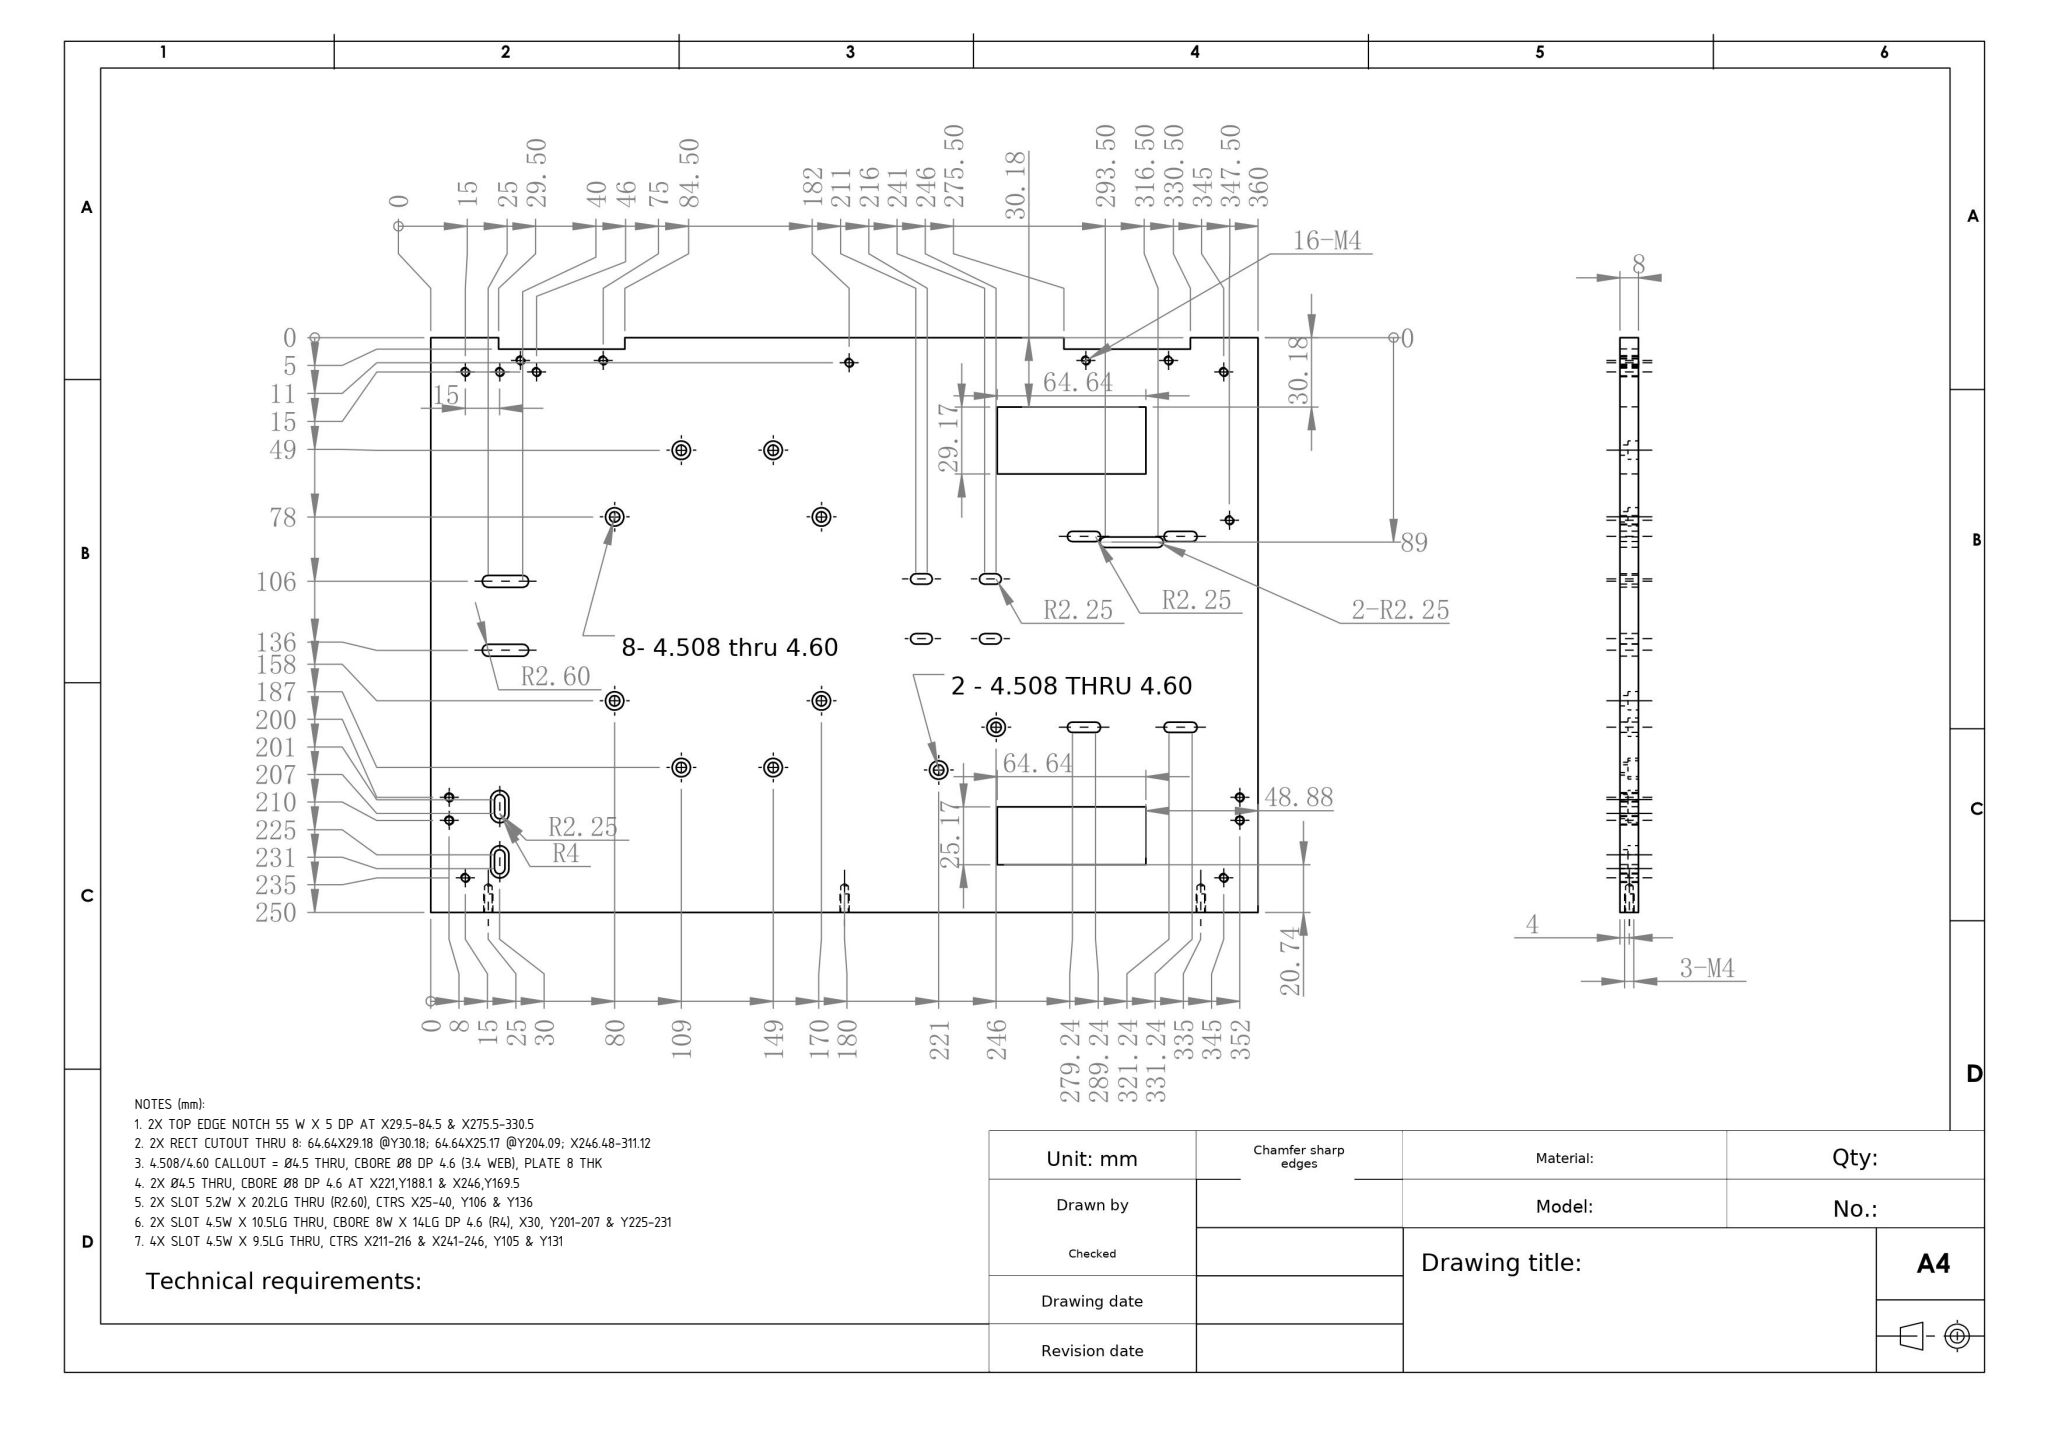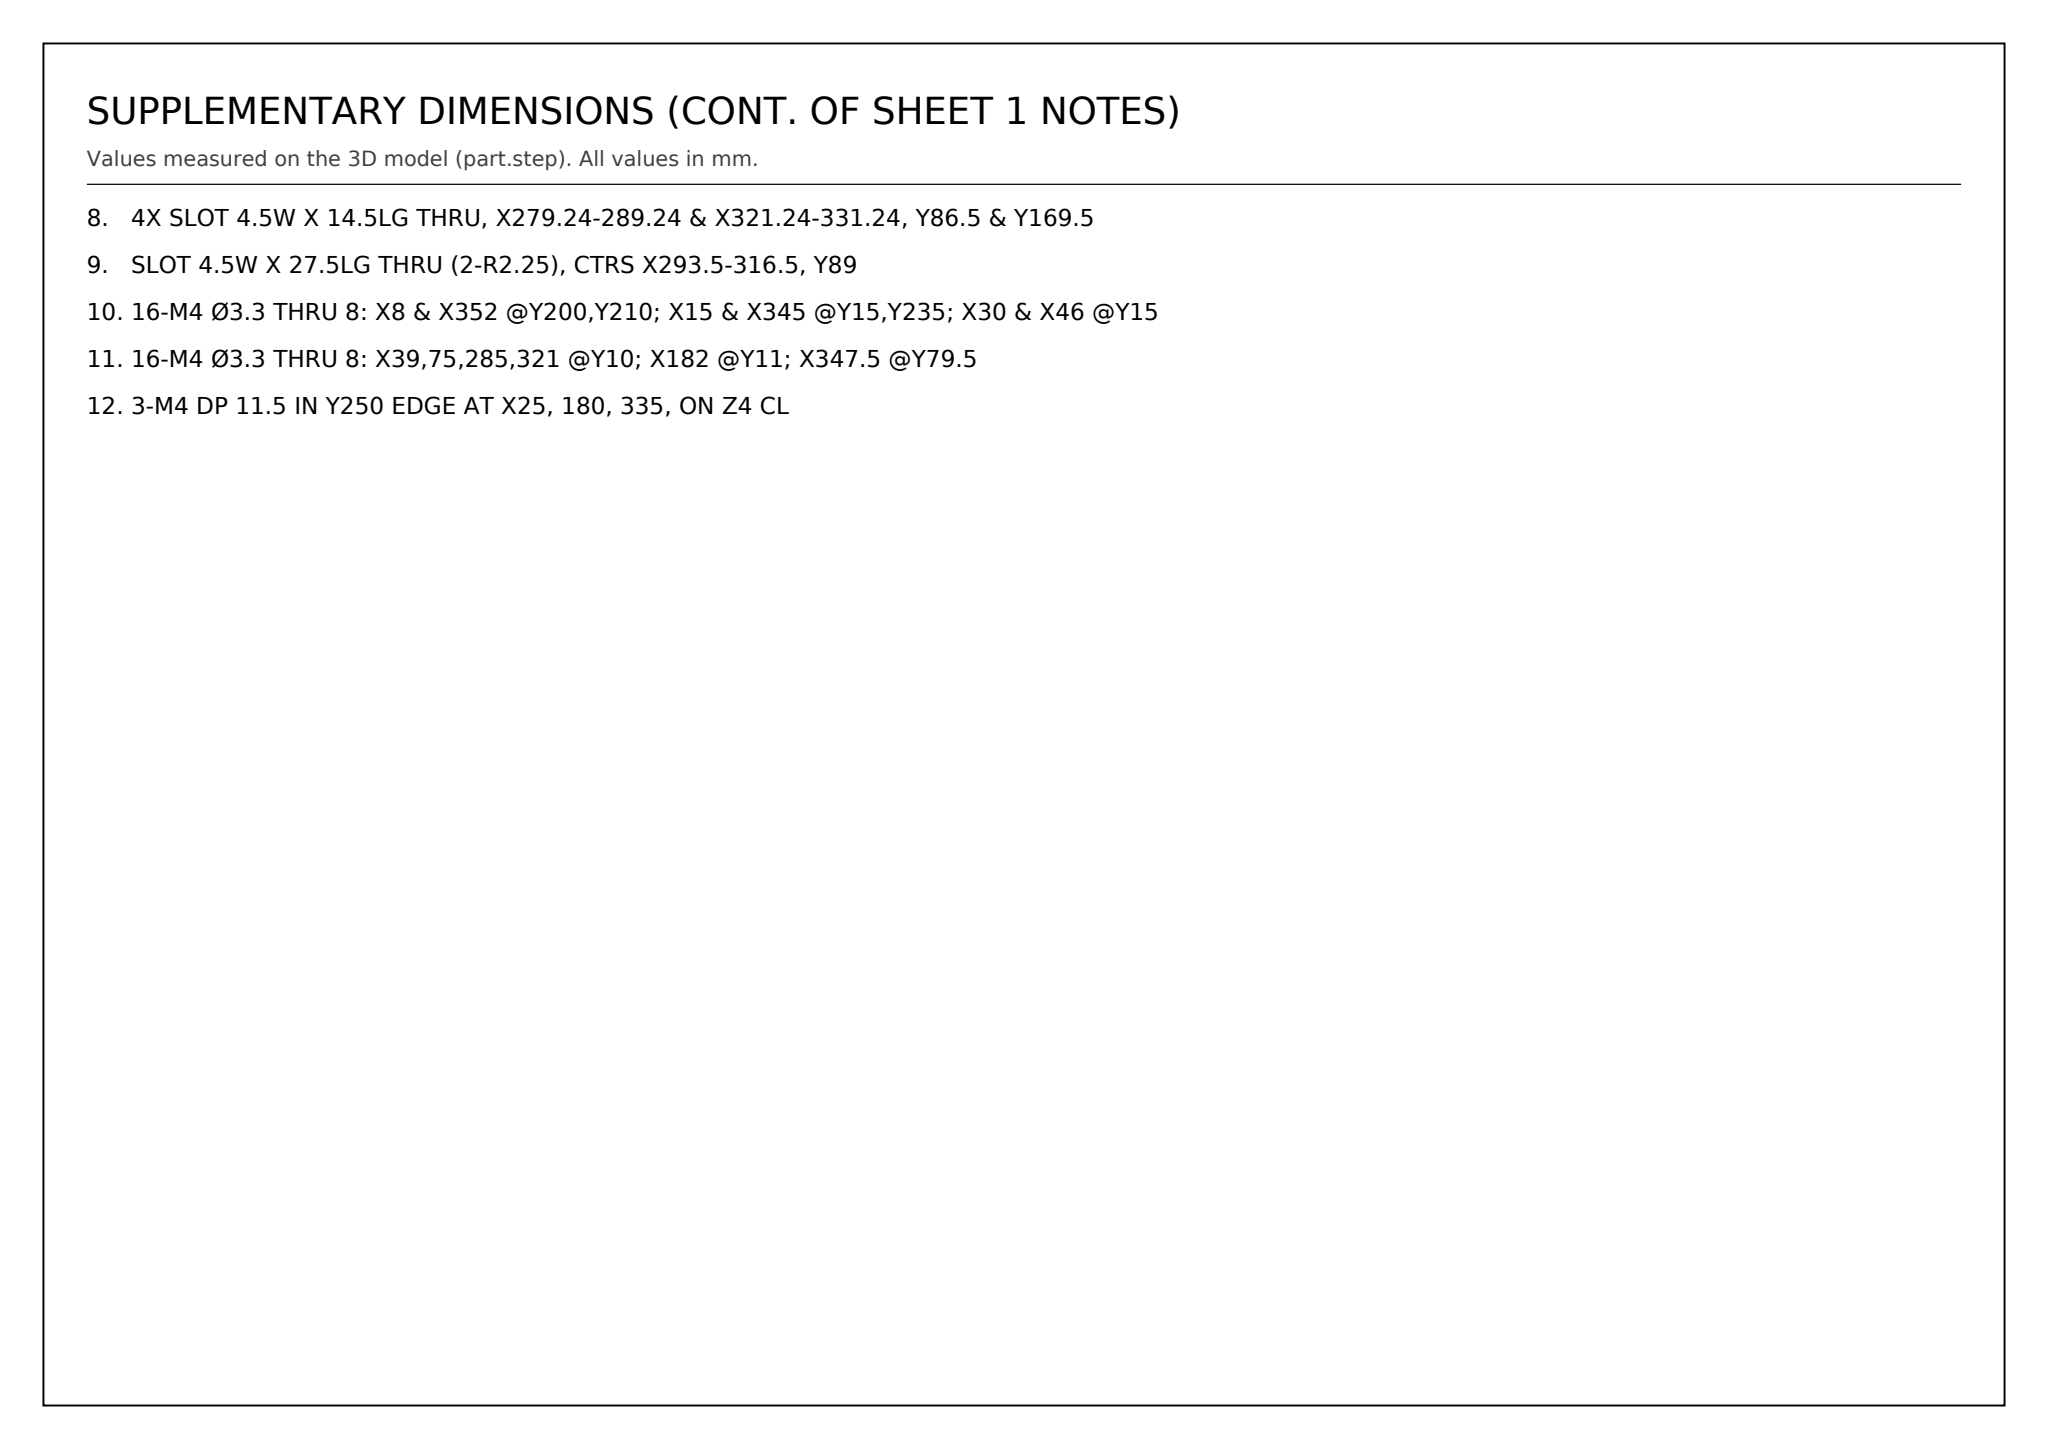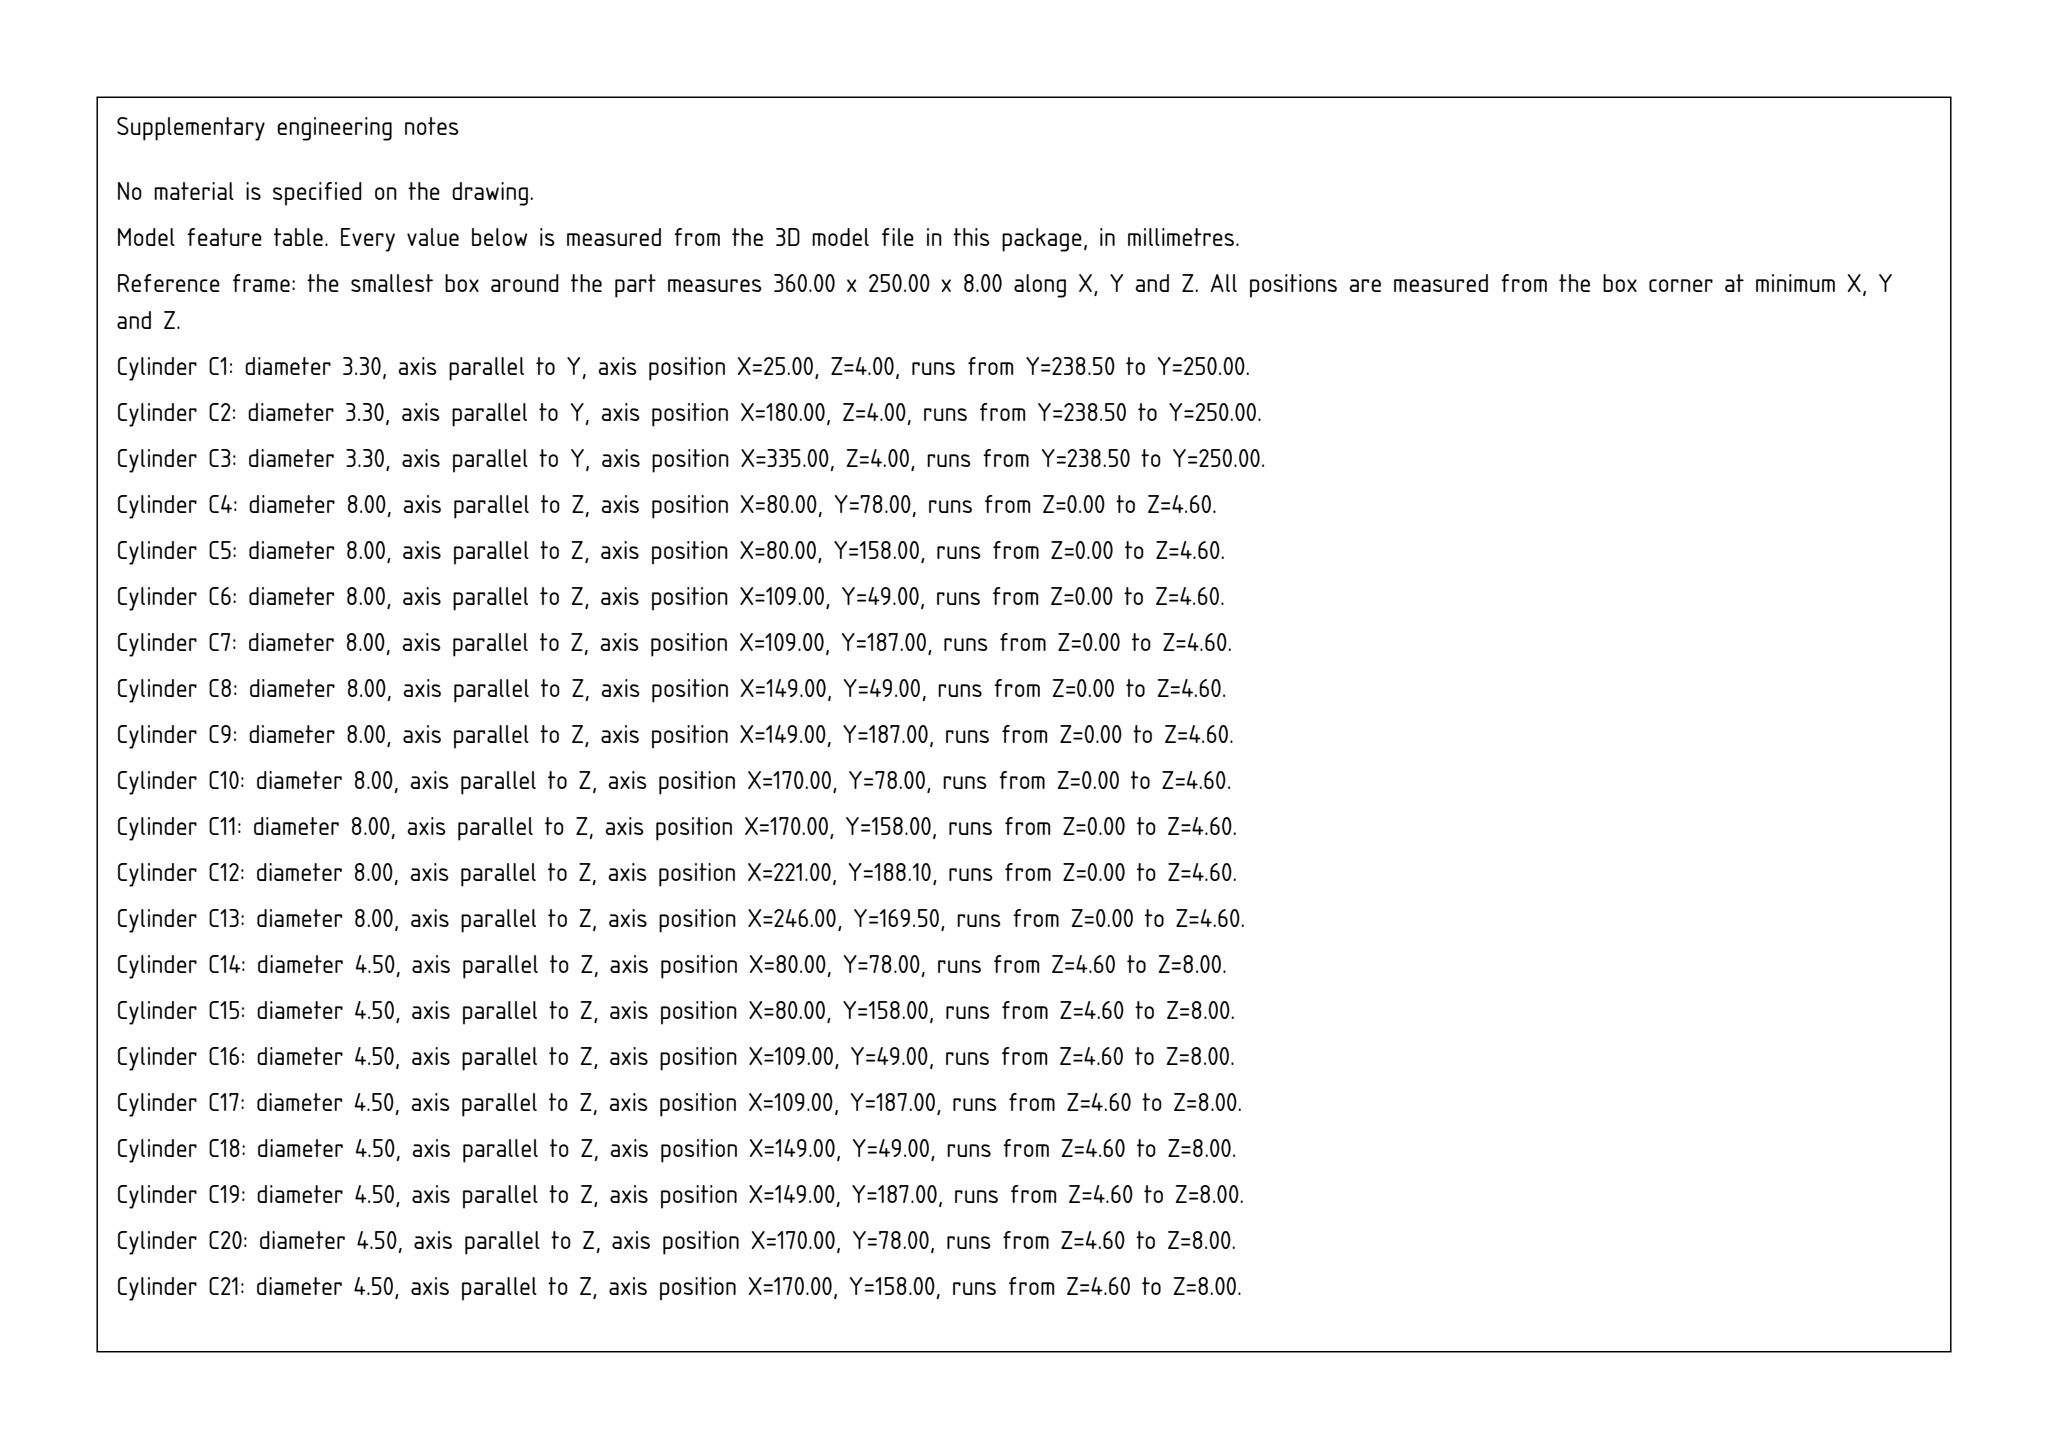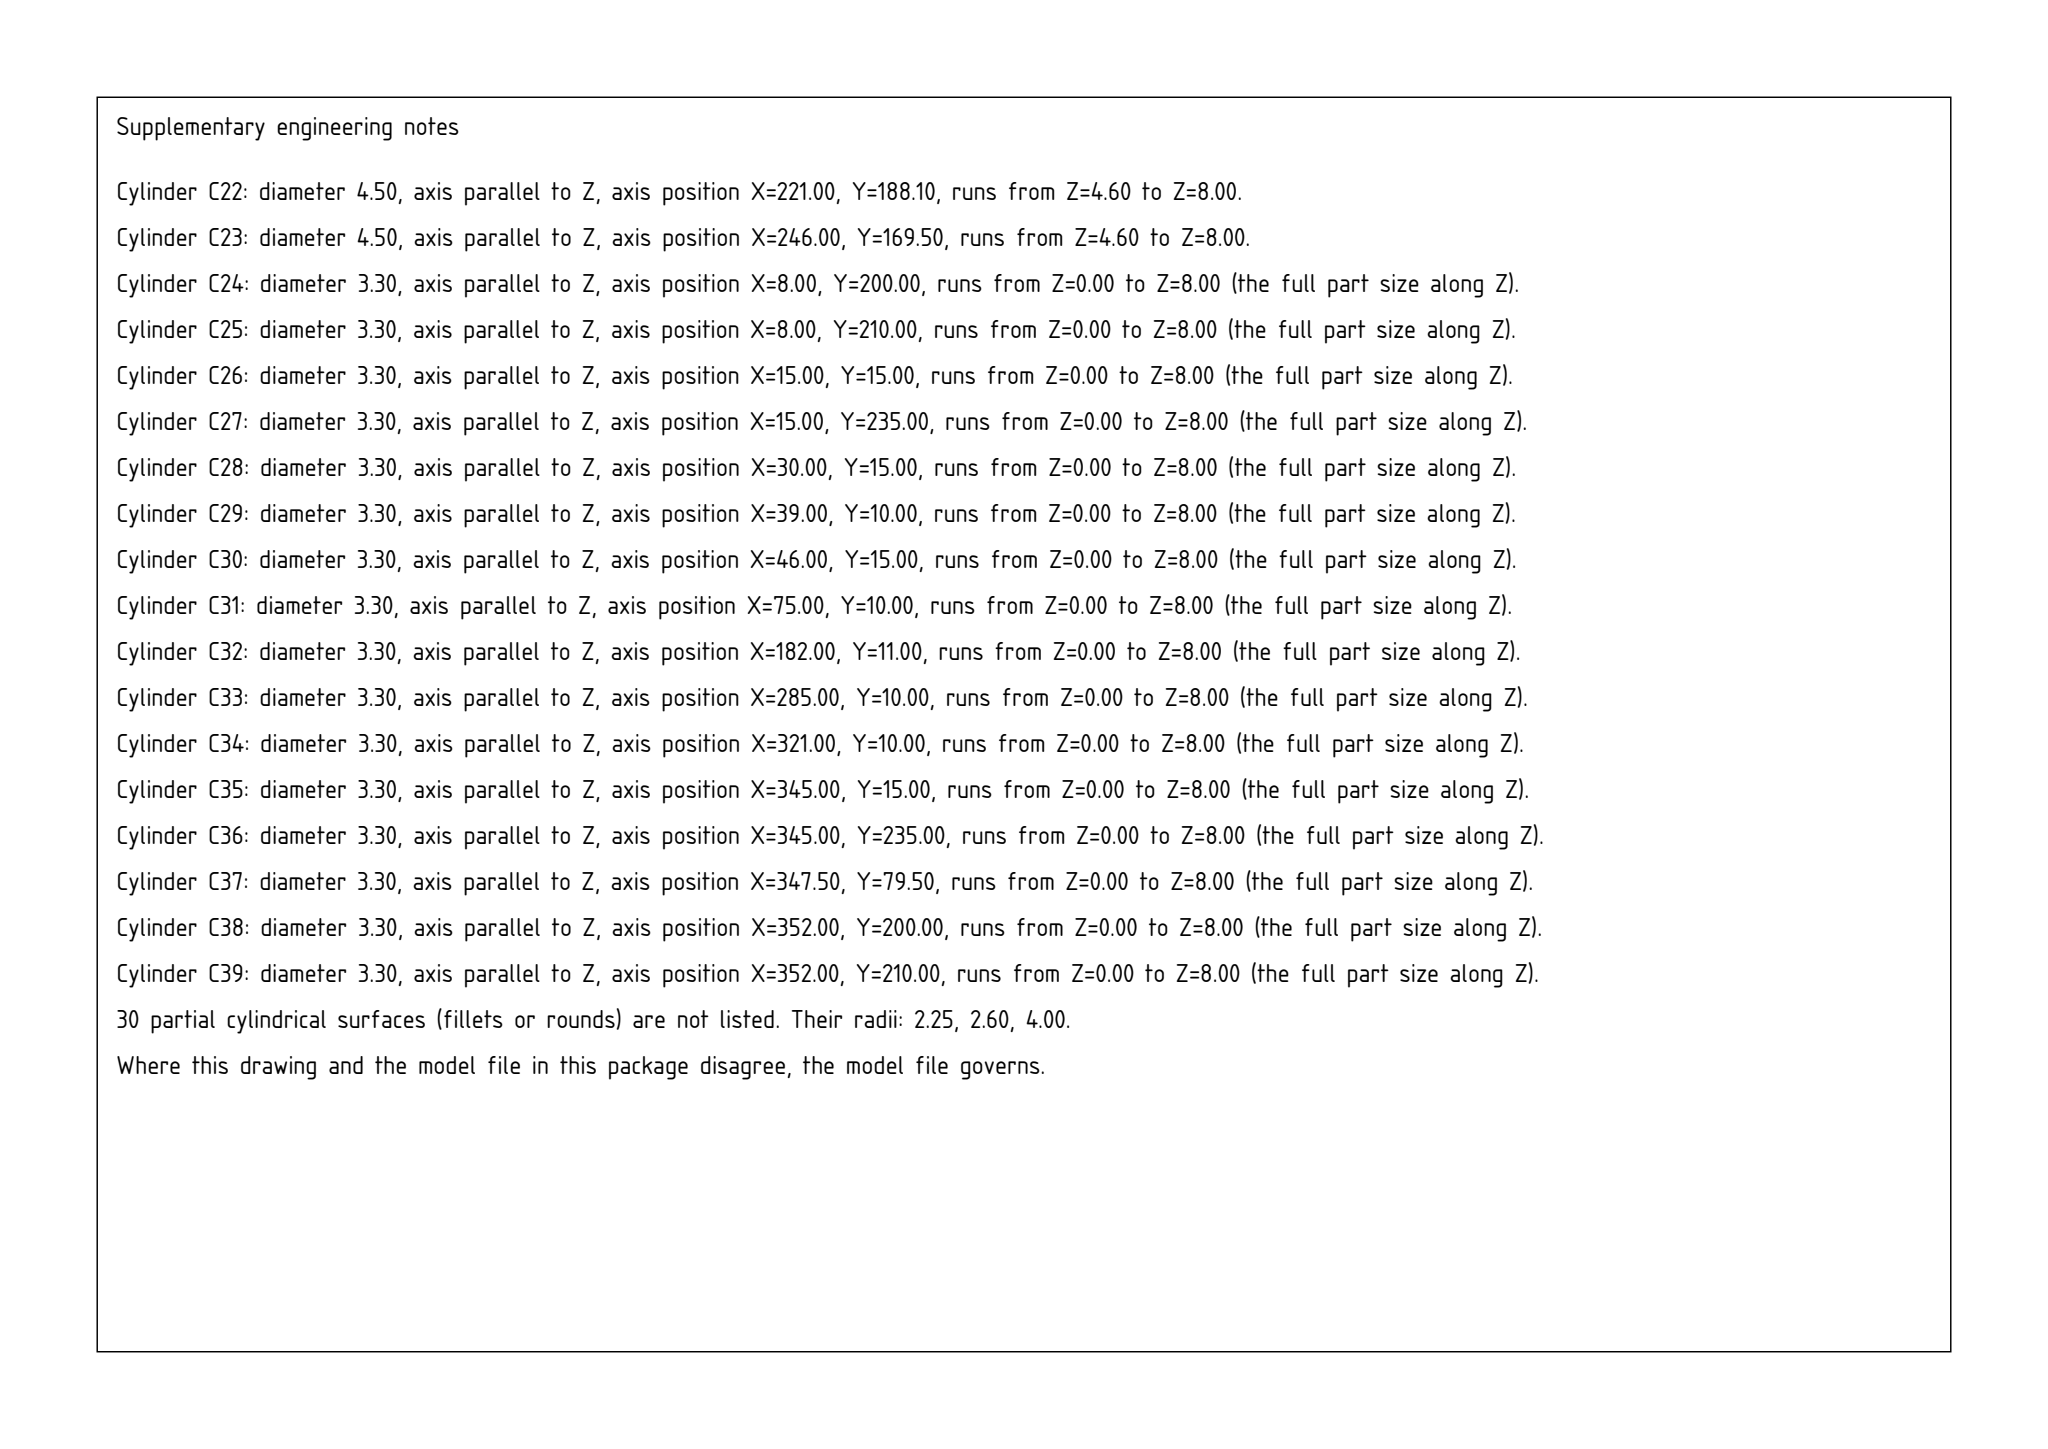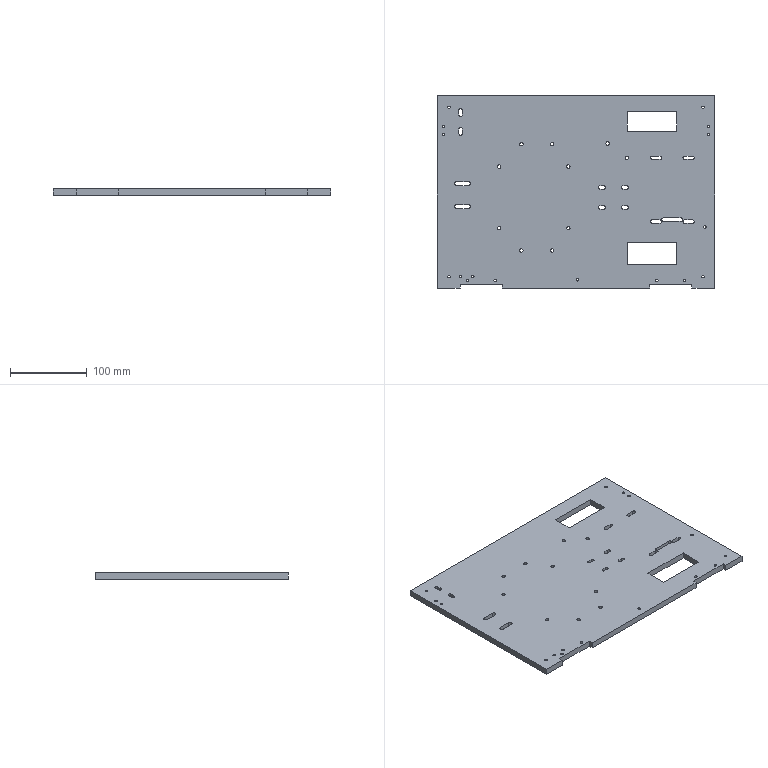Part | SolidWorks | mm | 1 solid | 189 faces | box 360 x 250 x 8 mm | volume 676328 mm3 | cylinder 119 | plane 64 | cone 6 | commonest cylinder face diameters 4.5 x51 3.3 x38 8 x24 5.2 x6
Drawing notes:
2X TOP EDGE NOTCH 55 W X 5 DP AT X29.5-84.5 & X275.5-330.5 | from the solid: x-planes 29.5/84.5/275.5/330.5 (55 apart); y-plane 5.0 count 2 offset from top edge y=0
2X RECT CUTOUT THRU 8: 64.64X29.18 @Y30.18; 64.64X25.17 @Y204.09; X246.48-311.12 | from the solid: x-planes 246.48 & 311.12; y 30.18/59.36=29.18, 204.09/229.26=25.17; z-planes only 0/4.6(cbore)/8
4.508/4.60 CALLOUT = Ø4.5 THRU, CBORE Ø8 DP 4.6 (3.4 WEB), PLATE 8 THK | from the solid: Ø4.5 cyl L=3.4 coaxial with Ø8.0 cyl L=4.6 same XY; 3.4+4.6=8.0=bbox Z; z-plane 4.6 x12
2X Ø4.5 THRU, CBORE Ø8 DP 4.6 AT X221,Y188.1 & X246,Y169.5 | from the solid: Ø4.5 L=3.4 + Ø8.0 L=4.6 at (221,188.1) and (246,169.5)
2X SLOT 5.2W X 20.2LG THRU (R2.60), CTRS X25-40, Y106 & Y136 | from the solid: Ø5.2 z-cyl L=8.0 at (25,106)(40,106)(25,136)(40,136); ctr dist 15
2X SLOT 4.5W X 10.5LG THRU, CBORE 8W X 14LG DP 4.6 (R4), X30, Y201-207 & Y225-231 | from the solid: Ø4.5 L3.4 + Ø8.0 L4.6 at (30,201)(30,207)(30,225)(30,231); ctr dist 6
4X SLOT 4.5W X 9.5LG THRU, CTRS X211-216 & X241-246, Y105 & Y131 | from the solid: Ø4.5 z-cyl L=8.0 at (211,105)(216,105)(241,105)(246,105) and same X @Y131
4X SLOT 4.5W X 14.5LG THRU, X279.24-289.24 & X321.24-331.24, Y86.5 & Y169.5 | from the solid: Ø4.5 z-cyl L=8.0 at x279.24/289.24/321.24/331.24, y86.5 & 169.5; ctr dist 10
SLOT 4.5W X 27.5LG THRU (2-R2.25), CTRS X293.5-316.5, Y89 | from the solid: Ø4.5 z-cyl L=8.0 at (293.5,89) and (316.5,89); ctr dist 23
16-M4 Ø3.3 THRU 8: X8 & X352 @Y200,Y210; X15 & X345 @Y15,Y235; X30 & X46 @Y15 | from the solid: Ø3.3 z-thru holes L=8 at (8,200)(8,210)(352,200)(352,210)(15,15)(15,235)(345,15)(345,235)(30,15)(46,15)
16-M4 Ø3.3 THRU 8: X39,75,285,321 @Y10; X182 @Y11; X347.5 @Y79.5 | from the solid: Ø3.3 z-thru holes L=8 at (39,10)(75,10)(285,10)(321,10)(182,11)(347.5,79.5)
3-M4 DP 11.5 IN Y250 EDGE AT X25, 180, 335, ON Z4 CL | from the solid: Ø3.3 y-axis cyl L=11.5 at x=25,180,335, z=4.0; 118 deg drill point
build123d program:
from build123d import *

# Parameters (mm, degrees)
SKETCH1_W                                            = 360
SKETCH1_H                                            = 250
BOSS_EXTRUDE1_DEPTH                                  = 8
HOLE_SIZE_ACCORDING_TO_HEXAGON_SOCKET_HE_D           = 4.5
HOLE_SIZE_ACCORDING_TO_HEXAGON_SOCKET_HE_CBORE_D     = 8
HOLE_SIZE_ACCORDING_TO_HEXAGON_SOCKET_HE_CBORE_DEPTH = 4.6
CUT_EXTRUDE1_DEPTH                                   = 10
CUT_EXTRUDE2_DEPTH                                   = 10
M4_TAPPED_HOLE3_D                                    = 3.3
M4_TAPPED_HOLE3_DEPTH                                = 21.5
M4_TAPPED_HOLE3_TIP                                  = 0.9914
M4_TAPPED_HOLE4_D                                    = 3.3
M4_TAPPED_HOLE4_DEPTH                                = 21.5
M4_TAPPED_HOLE4_TIP                                  = 0.9914
M4_TAPPED_HOLE5_D                                    = 3.3
M4_TAPPED_HOLE5_DEPTH                                = 11.5
M4_TAPPED_HOLE5_TIP                                  = 0.9914
M4_TAPPED_HOLE6_D                                    = 3.3
M4_TAPPED_HOLE6_DEPTH                                = 10.1
M4_TAPPED_HOLE6_TIP                                  = 0.9914
SKETCH22_W                                           = 55
SKETCH22_H                                           = 5
CUT_EXTRUDE3_DEPTH                                   = 10
M4_TAPPED_HOLE10_D                                   = 3.3
M4_TAPPED_HOLE10_DEPTH                               = 11.5
M4_TAPPED_HOLE10_TIP                                 = 0.9914
M4_TAPPED_HOLE11_D                                   = 3.3
M4_TAPPED_HOLE11_DEPTH                               = 11.5
M4_TAPPED_HOLE11_TIP                                 = 0.9914
CUT_EXTRUDE4_DEPTH                                   = 10
CUT_EXTRUDE5_DEPTH                                   = 10
M4_TAPPED_HOLE12_D                                   = 3.3
M4_TAPPED_HOLE12_DEPTH                               = 11.5
M4_TAPPED_HOLE12_TIP                                 = 0.9914
HOLE_SIZE_ACCORDING_TO_HEXAGON_SOCKE_2_D             = 4.5
HOLE_SIZE_ACCORDING_TO_HEXAGON_SOCKE_2_CBORE_D       = 8
HOLE_SIZE_ACCORDING_TO_HEXAGON_SOCKE_2_CBORE_DEPTH   = 4.6
CUT_EXTRUDE7_DEPTH                                   = 10
SKETCH38_W                                           = 64.642
SKETCH38_H                                           = 25.17
SKETCH38_H_2                                         = 29.175
CUT_EXTRUDE8_DEPTH                                   = 306


with BuildPart() as part:
    # Sketch1 → Boss-Extrude1 (new body)
    with BuildSketch(Plane.XY):
        with Locations((180, 125)):
            Rectangle(SKETCH1_W, SKETCH1_H)
    extrude(amount=BOSS_EXTRUDE1_DEPTH)

    # Hole Size according to Hexagon Socket He (through all)
    with Locations(Plane(origin=(0, 0, 0), x_dir=(-1, 0, 0), z_dir=(0, 0, -1))):
        with Locations((-30, 204), (-30, 228), (-149, 187), (-109, 187), (-170, 158), (-170, 78), (-149, 49), (-109, 49), (-80, 78), (-80, 158)):
            CounterBoreHole(HOLE_SIZE_ACCORDING_TO_HEXAGON_SOCKET_HE_D / 2, HOLE_SIZE_ACCORDING_TO_HEXAGON_SOCKET_HE_CBORE_D / 2, HOLE_SIZE_ACCORDING_TO_HEXAGON_SOCKET_HE_CBORE_DEPTH)

    # Sketch4 → Cut-Extrude1 (cut)
    with BuildSketch(Plane(origin=(0, 0, 0), x_dir=(-1, 0, 0), z_dir=(0, 0, -1))):
        with BuildLine():
            Line((-289.238, 88.75), (-279.238, 88.75))
            ThreePointArc((-279.238, 88.75), (-276.988, 86.5), (-279.238, 84.25))
            Line((-279.238, 84.25), (-289.238, 84.25))
            ThreePointArc((-289.238, 84.25), (-291.488, 86.5), (-289.238, 88.75))
        make_face()
        with BuildLine():
            Line((-331.238, 84.25), (-321.238, 84.25))
            ThreePointArc((-321.238, 84.25), (-318.988, 86.5), (-321.238, 88.75))
            Line((-321.238, 88.75), (-331.238, 88.75))
            ThreePointArc((-331.238, 88.75), (-333.488, 86.5), (-331.238, 84.25))
        make_face()
        with BuildLine():
            Line((-331.238, 171.75), (-321.238, 171.75))
            ThreePointArc((-321.238, 171.75), (-318.988, 169.5), (-321.238, 167.25))
            Line((-321.238, 167.25), (-331.238, 167.25))
            ThreePointArc((-331.238, 167.25), (-333.488, 169.5), (-331.238, 171.75))
        make_face()
        with BuildLine():
            Line((-289.238, 167.25), (-279.238, 167.25))
            ThreePointArc((-279.238, 167.25), (-276.988, 169.5), (-279.238, 171.75))
            Line((-279.238, 171.75), (-289.238, 171.75))
            ThreePointArc((-289.238, 171.75), (-291.488, 169.5), (-289.238, 167.25))
        make_face()
        with BuildLine():
            Line((-40, 108.6), (-25, 108.6))
            ThreePointArc((-25, 108.6), (-22.4, 106), (-25, 103.4))
            Line((-25, 103.4), (-40, 103.4))
            ThreePointArc((-40, 103.4), (-42.6, 106), (-40, 108.6))
        make_face()
        with BuildLine():
            Line((-40, 138.6), (-25, 138.6))
            ThreePointArc((-25, 138.6), (-22.4, 136), (-25, 133.4))
            Line((-25, 133.4), (-40, 133.4))
            ThreePointArc((-40, 133.4), (-42.6, 136), (-40, 138.6))
        make_face()
    extrude(amount=-CUT_EXTRUDE1_DEPTH, mode=Mode.SUBTRACT)

    # Sketch7 → Cut-Extrude2 (cut)
    with BuildSketch(Plane.XY.offset(8)):
        with BuildLine():
            Line((241, 133.25), (246, 133.25))
            ThreePointArc((246, 133.25), (248.25, 131), (246, 128.75))
            Line((246, 128.75), (241, 128.75))
            ThreePointArc((241, 128.75), (238.75, 131), (241, 133.25))
        make_face()
        with BuildLine():
            Line((211, 107.25), (216, 107.25))
            ThreePointArc((216, 107.25), (218.25, 105), (216, 102.75))
            Line((216, 102.75), (211, 102.75))
            ThreePointArc((211, 102.75), (208.75, 105), (211, 107.25))
        make_face()
        with BuildLine():
            Line((211, 133.25), (216, 133.25))
            ThreePointArc((216, 133.25), (218.25, 131), (216, 128.75))
            Line((216, 128.75), (211, 128.75))
            ThreePointArc((211, 128.75), (208.75, 131), (211, 133.25))
        make_face()
        with BuildLine():
            Line((241, 107.25), (246, 107.25))
            ThreePointArc((246, 107.25), (248.25, 105), (246, 102.75))
            Line((246, 102.75), (241, 102.75))
            ThreePointArc((241, 102.75), (238.75, 105), (241, 107.25))
        make_face()
    extrude(amount=-CUT_EXTRUDE2_DEPTH, mode=Mode.SUBTRACT)

    # M4 Tapped Hole3
    with Locations(Plane.XY.offset(8)):
        with Locations((182, 11), (347.5, 79.5)):
            Hole(M4_TAPPED_HOLE3_D / 2, depth=M4_TAPPED_HOLE3_DEPTH)
            with Locations((0, 0, -(M4_TAPPED_HOLE3_DEPTH + M4_TAPPED_HOLE3_TIP / 2))):  # 118° drill point
                Cone(0, M4_TAPPED_HOLE3_D / 2, M4_TAPPED_HOLE3_TIP, mode=Mode.SUBTRACT)

    # M4 Tapped Hole4
    with Locations(Plane.XY.offset(8)):
        with Locations((15, 235), (15, 15), (345, 15), (345, 235)):
            Hole(M4_TAPPED_HOLE4_D / 2, depth=M4_TAPPED_HOLE4_DEPTH)
            with Locations((0, 0, -(M4_TAPPED_HOLE4_DEPTH + M4_TAPPED_HOLE4_TIP / 2))):  # 118° drill point
                Cone(0, M4_TAPPED_HOLE4_D / 2, M4_TAPPED_HOLE4_TIP, mode=Mode.SUBTRACT)

    # M4 Tapped Hole5
    with Locations(Plane.XY.offset(8)):
        with Locations((246, 169.5), (221, 188.1)):
            Hole(M4_TAPPED_HOLE5_D / 2, depth=M4_TAPPED_HOLE5_DEPTH)
            with Locations((0, 0, -(M4_TAPPED_HOLE5_DEPTH + M4_TAPPED_HOLE5_TIP / 2))):  # 118° drill point
                Cone(0, M4_TAPPED_HOLE5_D / 2, M4_TAPPED_HOLE5_TIP, mode=Mode.SUBTRACT)

    # M4 Tapped Hole6
    with Locations(Plane.XY.offset(8)):
        with Locations((46, 15), (30, 15)):
            Hole(M4_TAPPED_HOLE6_D / 2, depth=M4_TAPPED_HOLE6_DEPTH)
            with Locations((0, 0, -(M4_TAPPED_HOLE6_DEPTH + M4_TAPPED_HOLE6_TIP / 2))):  # 118° drill point
                Cone(0, M4_TAPPED_HOLE6_D / 2, M4_TAPPED_HOLE6_TIP, mode=Mode.SUBTRACT)

    # Sketch22 → Cut-Extrude3 (cut)
    with BuildSketch(Plane.XY.offset(8)):
        with Locations((303, 2.5)):
            Rectangle(SKETCH22_W, SKETCH22_H)
        with Locations((57, 2.5)):
            Rectangle(SKETCH22_W, SKETCH22_H)
    extrude(amount=-CUT_EXTRUDE3_DEPTH, mode=Mode.SUBTRACT)

    # M4 Tapped Hole10
    with Locations(Plane.XY.offset(8)):
        with Locations((39, 10), (75, 10), (285, 10), (321, 10)):
            Hole(M4_TAPPED_HOLE10_D / 2, depth=M4_TAPPED_HOLE10_DEPTH)
            with Locations((0, 0, -(M4_TAPPED_HOLE10_DEPTH + M4_TAPPED_HOLE10_TIP / 2))):  # 118° drill point
                Cone(0, M4_TAPPED_HOLE10_D / 2, M4_TAPPED_HOLE10_TIP, mode=Mode.SUBTRACT)

    # M4 Tapped Hole11
    with Locations(Plane(origin=(0, 0, 0), x_dir=(-1, 0, 0), z_dir=(0, 0, -1))):
        with Locations((-8, 210), (-8, 200), (-352, 210), (-352, 200)):
            Hole(M4_TAPPED_HOLE11_D / 2, depth=M4_TAPPED_HOLE11_DEPTH)
            with Locations((0, 0, -(M4_TAPPED_HOLE11_DEPTH + M4_TAPPED_HOLE11_TIP / 2))):  # 118° drill point
                Cone(0, M4_TAPPED_HOLE11_D / 2, M4_TAPPED_HOLE11_TIP, mode=Mode.SUBTRACT)

    # Sketch29 → Cut-Extrude4 (cut)
    with BuildSketch(Plane(origin=(0, 0, 4.6), x_dir=(-1, 0, 0), z_dir=(0, 0, -1))):
        with BuildLine():
            Line((-27.75, 231), (-27.75, 225))
            ThreePointArc((-27.75, 225), (-30, 222.75), (-32.25, 225))
            Line((-32.25, 225), (-32.25, 231))
            ThreePointArc((-32.25, 231), (-30, 233.25), (-27.75, 231))
        make_face()
        with BuildLine():
            Line((-32.25, 201), (-32.25, 207))
            ThreePointArc((-32.25, 207), (-30, 209.25), (-27.75, 207))
            Line((-27.75, 207), (-27.75, 201))
            ThreePointArc((-27.75, 201), (-30, 198.75), (-32.25, 201))
        make_face()
    extrude(amount=-CUT_EXTRUDE4_DEPTH, mode=Mode.SUBTRACT)

    # Sketch30 → Cut-Extrude5 (cut)
    with BuildSketch(Plane.XY.offset(4.6)):
        with BuildLine():
            Line((34, 231), (34, 225))
            ThreePointArc((34, 225), (30, 221), (26, 225))
            Line((26, 225), (26, 231))
            ThreePointArc((26, 231), (30, 235), (34, 231))
        make_face()
        with BuildLine():
            Line((26, 201), (26, 207))
            ThreePointArc((26, 207), (30, 211), (34, 207))
            Line((34, 207), (34, 201))
            ThreePointArc((34, 201), (30, 197), (26, 201))
        make_face()
    extrude(amount=-CUT_EXTRUDE5_DEPTH, mode=Mode.SUBTRACT)

    # M4 Tapped Hole12
    with Locations(Plane(origin=(0, 250, 0), x_dir=(-1, 0, 0), z_dir=(0, 1, 0))):
        with Locations((-25, 4), (-180, 4), (-335, 4)):
            Hole(M4_TAPPED_HOLE12_D / 2, depth=M4_TAPPED_HOLE12_DEPTH)
            with Locations((0, 0, -(M4_TAPPED_HOLE12_DEPTH + M4_TAPPED_HOLE12_TIP / 2))):  # 118° drill point
                Cone(0, M4_TAPPED_HOLE12_D / 2, M4_TAPPED_HOLE12_TIP, mode=Mode.SUBTRACT)

    # Hole Size according to Hexagon Socke 2 (through all)
    with Locations(Plane(origin=(0, 0, 0), x_dir=(-1, 0, 0), z_dir=(0, 0, -1))):
        with Locations((-221, 188.1), (-246, 169.5)):
            CounterBoreHole(HOLE_SIZE_ACCORDING_TO_HEXAGON_SOCKE_2_D / 2, HOLE_SIZE_ACCORDING_TO_HEXAGON_SOCKE_2_CBORE_D / 2, HOLE_SIZE_ACCORDING_TO_HEXAGON_SOCKE_2_CBORE_DEPTH)

    # Sketch37 → Cut-Extrude7 (cut)
    with BuildSketch(Plane(origin=(0, 0, 0), x_dir=(-1, 0, 0), z_dir=(0, 0, -1))):
        with BuildLine():
            Line((-316.5, 91.25), (-293.5, 91.25))
            ThreePointArc((-293.5, 91.25), (-291.25, 89), (-293.5, 86.75))
            Line((-293.5, 86.75), (-316.5, 86.75))
            ThreePointArc((-316.5, 86.75), (-318.75, 89), (-316.5, 91.25))
        make_face()
    extrude(amount=-CUT_EXTRUDE7_DEPTH, mode=Mode.SUBTRACT)

    # Sketch38 → Cut-Extrude8 (cut)
    with BuildSketch(Plane(origin=(0, 0, 0), x_dir=(-1, 0, 0), z_dir=(0, 0, -1))):
        with Locations((-278.8, 216.671)):
            Rectangle(SKETCH38_W, SKETCH38_H)
        with Locations((-278.8, 44.77)):
            Rectangle(SKETCH38_W, SKETCH38_H_2)
    extrude(amount=-CUT_EXTRUDE8_DEPTH, mode=Mode.SUBTRACT)


solid = part.part